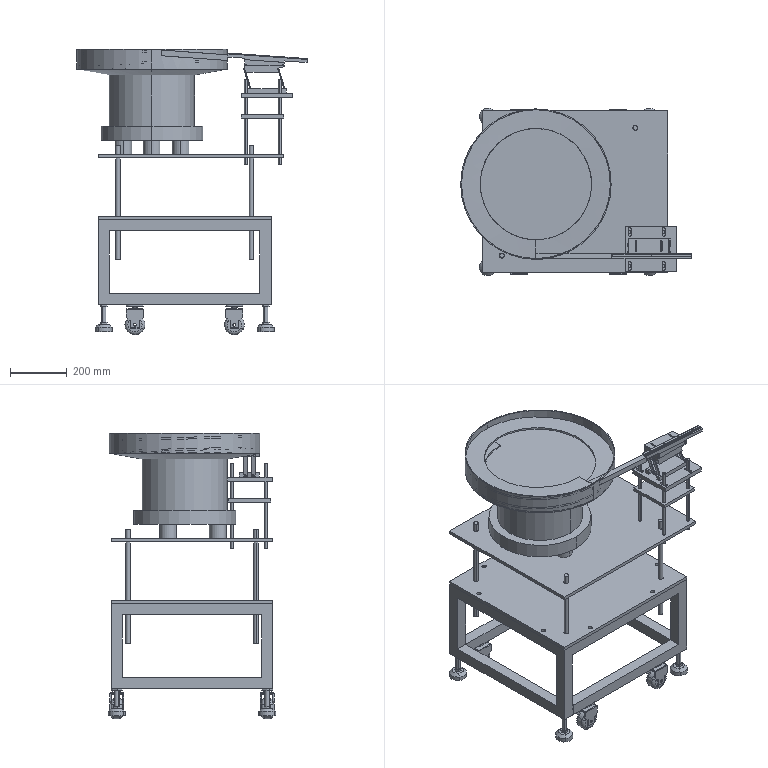Assembly | SolidWorks | mm | 52 component files | 52 solids | 1070 faces | box 812.32 x 590 x 1004.72 mm | volume 42903863 mm3 | plane 672 | cylinder 321 | cone 58 | torus 16 | spline 3 | commonest cylinder face diameters 10 x56 16 x40 10.5 x24 15 x16 9 x16 6.5 x16 3.3 x16 4.5 x16
Bill of materials:
Wheel | 4 |  | Short solid cylinder with large rounded edges on both ends and a small central axial hole.
WheelBracket | 4 |  | U-shaped bent-sheet bracket: a flat rectangular top web with one small hole, and two parallel side flanges folded down. Each flange narrows to a lower tab with one round hole.
WheelRetainingBlock | 4 |  | Flat plate shaped like a rectangle with rounded ends. It has one larger central hole and two smaller holes, one at each end on the long axis, plus a protrusion on the underside with a curved/tapered profile.
WheelRetainingPin | 4 |  | Plain solid cylinder with small chamfers on both end edges.
FootPad | 4 |  | Turned part: a slender cylindrical shaft rising from a larger short cylindrical base. The base has a conical chamfer between its outer edge and the shaft.
FootPadScrew | 8 |  | Hexagonal ring/nut-like body with a large round central bore and chamfered corners on both faces.
Frame01-1 | 1 |  | Open rectangular box frame made of square-section members along all twelve edges of a rectangular prism.
CSFA2082 072 | 1 |  | Thin flat rectangular (near-square) plate with twelve through holes around the perimeter: four larger holes inset at the corners and eight smaller holes in pairs along each edge.
CSFA2082 073 | 1 |  | Thin flat rectangular plate with four larger holes near the corners and four smaller holes in a square pattern around one of the corner holes.
CSFA2082 074 | 1 |  | Square flat plate of moderate thickness with four through holes, one inset near each corner.
CSFA2082 076 | 1 |  | Thick rectangular plate with four elongated slots near the corners, all running the same direction, and a faint thin L-shaped line or groove on the top face.
CSFA2082 077 | 1 |  | Rectangular block shaped like a wedge, with a top face sloping along its length. It has four larger holes at the corners and four smaller holes inboard in two pairs.
CSFA2082 078-1 | 4 |  | Long, slender, straight solid-looking cylindrical rod with flat ends.
CSFA2082 078 | 4 |  | Long, slender, straight cylindrical rod with flat ends, nearly identical to unnamed part but slightly thicker relative to its length.
CSFA2082 079 | 1 |  | Long, narrow base strip with a wider rectangular plate section in the middle on one side. A lengthwise rectangular channel runs along the strip, the plate section has two parallel elongated slots, and small round holes are spaced along the strip.
FeedingPressureBlock | 2 |  | Thin, flat rectangular bar with two round holes spaced along its length.
Part77 | 1 |  | Rectangular block or plate with angled long side faces and a notched, angled profile at one end. Several round holes are grouped near each short end, with one near the centre.
Part78 | 1 |  | Thick rectangular plate with a rectangular notch centred in each short end, leaving four corner ears. Each ear has one round hole.
Part79 | 4 |  | Flat rectangular link bar with square ends and one round hole near each end.
PlasticVibratoryFeederCSFA2082 | 1 |  | Rotationally symmetric part: a large disc head with a conical underside, a narrower cylindrical body, a flange ring below, and small cylindrical pins sticking out of the bottom. A shallow circular groove is on the top face, and a thin radial strip or tab extends past the head's rim.
Mates:
1. concentric | CSFA2082 072-1 face at (132.551, 208.824, 240) dir (0, 0, 1) r 8.5 | CSFA2082 073-1 face at (132.551, 208.824, 457) dir (0, 0, 1) r 9
2. distance | CSFA2082 072-1 face at (202.551, 268.824, 240) dir (0, 0, 1) | CSFA2082 073-1 face at (247.551, 268.824, 445) dir (0, 0, -1)
3. coincident | CSFA2082 073-1 face at (247.551, 268.824, 457) dir (0, 0, 1) | PlasticVibratoryFeederCSFA2082-1 face at (-217.593, -107.346, 457) dir (0, 0, -1)
4. distance | CSFA2082 074-1 face at (247.551, -143.176, 585) dir (0, 0, -1) | CSFA2082 073-1 face at (247.551, 268.824, 457) dir (0, 0, 1)
5. coincident | CSFA2082 076-1 face at (277.301, -138.176, 673) dir (0, 0, 1) | FlatFeed-1/Part78-1 face at (256.301, -253.176, 673) dir (0, 0, -1)
6. coincident | FlatFeed-1/Part77-1 face at (248.594, -253.176, 771) dir (0, 0, 1) | CSFA2082 077-1 face at (248.594, -183.176, 771) dir (0, 0, -1)
7. concentric | CSFA2082 073-1 face at (132.551, -241.176, 457) dir (0, 0, 1) r 9 | CSFA2082 078-6 face at (132.551, -241.176, 487) dir (0, 0, -1) r 8
8. concentric | CSFA2082 073-1 face at (-337.449, -241.176, 457) dir (0, 0, 1) r 9 | CSFA2082 078-5 face at (-337.449, -241.176, 487) dir (0, 0, -1) r 8
9. concentric | CSFA2082 073-1 face at (-337.449, 208.824, 457) dir (0, 0, 1) r 9 | CSFA2082 078-9 face at (-337.449, 208.824, 487) dir (0, 0, -1) r 8
10. concentric | CSFA2082 073-1 face at (132.551, 208.824, 457) dir (0, 0, 1) r 9 | CSFA2082 078-7 face at (132.551, 208.824, 487) dir (0, 0, -1) r 8
11. coincident | CSFA2082 078-5 face at (-337.449, -241.176, 487) dir (0, 0, 1) | CSFA2082 078-6 face at (132.551, -241.176, 487) dir (0, 0, 1)
12. coincident | CSFA2082 078-5 face at (-337.449, -241.176, 487) dir (0, 0, 1) | CSFA2082 078-9 face at (-337.449, 208.824, 487) dir (0, 0, 1)
13. coincident | CSFA2082 078-5 face at (-337.449, -241.176, 487) dir (0, 0, 1) | CSFA2082 078-7 face at (132.551, 208.824, 487) dir (0, 0, 1)
14. coincident | CSFA2082 072-1 face at (202.551, 268.824, 228) dir (0, 0, -1) | AssemblyVibratoryFeederChassis-1/Frame01-1-1 face at (-407.449, 268.824, 228) dir (0, 0, 1)
15. concentric | CSFA2082 072-1 face at (-337.449, -241.176, 240) dir (0, 0, 1) r 8.5 | CSFA2082 078-5 face at (-337.449, -241.176, 487) dir (0, 0, -1) r 8
16. concentric | CSFA2082 073-1 face at (112.551, -278.176, 457) dir (0, 0, 1) r 5.25 | CSFA2082 078-1-1 face at (112.551, -278.176, 720) dir (0, 0, -1) r 5
17. concentric | CSFA2082 074-1 face at (112.551, -278.176, 597) dir (0, 0, 1) r 5.25 | CSFA2082 078-1-1 face at (112.551, -278.176, 720) dir (0, 0, -1) r 5
18. distance | CSFA2082 078-1-1 face at (112.551, -278.176, 420) dir (0, 0, -1) | CSFA2082 073-1 face at (247.551, 268.824, 445) dir (0, 0, -1)
19. concentric | CSFA2082 073-1 face at (232.551, -278.176, 457) dir (0, 0, 1) r 5.25 | CSFA2082 078-1-2 face at (232.551, -278.176, 720) dir (0, 0, -1) r 5
20. coincident | CSFA2082 078-1-1 face at (112.551, -278.176, 420) dir (0, 0, -1) | CSFA2082 078-1-2 face at (232.551, -278.176, 420) dir (0, 0, -1)
21. coincident | CSFA2082 078-1-2 face at (232.551, -278.176, 420) dir (0, 0, -1) | CSFA2082 078-1-4 face at (232.551, -158.176, 420) dir (0, 0, -1)
22. coincident | CSFA2082 078-1-3 face at (112.551, -158.176, 420) dir (0, 0, -1) | CSFA2082 078-1-4 face at (232.551, -158.176, 420) dir (0, 0, -1)
23. concentric | CSFA2082 073-1 face at (112.551, -158.176, 457) dir (0, 0, 1) r 5.25 | CSFA2082 078-1-3 face at (112.551, -158.176, 720) dir (0, 0, -1) r 5
24. concentric | CSFA2082 073-1 face at (232.551, -158.176, 457) dir (0, 0, 1) r 5.25 | CSFA2082 078-1-4 face at (232.551, -158.176, 720) dir (0, 0, -1) r 5
25. tangent | CSFA2082 076-1 face at (117.551, -268.176, 657) dir (-1, 0, 0) | CSFA2082 078-1-1 face at (112.551, -278.176, 720) dir (0, 0, -1) r 5
26. tangent | CSFA2082 076-1 face at (237.551, -268.176, 657) dir (-1, 0, 0) | CSFA2082 078-1-2 face at (232.551, -278.176, 720) dir (0, 0, -1) r 5
27. distance | CSFA2082 076-1 face at (97.301, -298.176, 673) dir (0, -1, 0) | CSFA2082 074-1 face at (97.551, -293.176, 597) dir (0, -1, 0)
28. distance | FlatFeed-1/Part78-1 face at (256.301, -253.176, 673) dir (0, -1, 0) | CSFA2082 076-1 face at (97.301, -298.176, 673) dir (0, -1, 0)
29. distance | CSFA2082 078-9 face at (-337.449, 208.824, 487) dir (0, 0, 1) | CSFA2082 073-1 face at (247.551, 268.824, 457) dir (0, 0, 1)
30. coincident | CSFA2082 079-1 face at (329.522, -253.176, 791.691) dir (0.06976, 0, 0.9976) | FeedingPressureBlock-1 face at (50.204, -233.176, 811.222) dir (-0.06976, 0, -0.9976)
31. concentric | CSFA2082 079-1 face at (85.119, -236.676, 808.781) dir (0.06976, 0, 0.9976) r 1.65 | FeedingPressureBlock-1 face at (85.328, -236.676, 811.774) dir (-0.06976, 0, -0.9976) r 2.25
32. concentric | CSFA2082 079-1 face at (154.949, -236.676, 803.898) dir (0.06976, 0, 0.9976) r 1.65 | FeedingPressureBlock-1 face at (155.158, -236.676, 806.891) dir (-0.06976, 0, -0.9976) r 2.25
33. distance | FlatFeed-1/Part78-1 face at (256.301, -253.176, 688) dir (1, 0, 0) | CSFA2082 076-1 face at (277.301, -298.176, 673) dir (1, 0, 0)
34. coincident | CSFA2082 079-1 face at (329.522, -253.176, 791.691) dir (0.06976, 0, 0.9976) | FeedingPressureBlock-2 face at (329.522, -233.176, 791.691) dir (-0.06976, 0, -0.9976)
35. concentric | CSFA2082 079-1 face at (224.778, -236.676, 799.015) dir (0.06976, 0, 0.9976) r 1.65 | FeedingPressureBlock-2 face at (224.778, -236.676, 799.015) dir (0.06976, 0, 0.9976) r 2.25
36. concentric | CSFA2082 079-1 face at (294.608, -236.676, 794.132) dir (0.06976, 0, 0.9976) r 1.65 | FeedingPressureBlock-2 face at (294.608, -236.676, 794.132) dir (0.06976, 0, 0.9976) r 2.25
37. coincident | PlasticVibratoryFeederCSFA2082-1 face at (-217.593, -253.176, 507) dir (0, -1, 0) | CSFA2082 079-1 face at (248.943, -253.176, 786.198) dir (0, -1, 0)
38. coincident | FlatFeed-1/Part77-1 face at (108.594, -253.176, 771) dir (-1, 0, 0) | CSFA2082 077-1 face at (108.594, -253.176, 791) dir (-1, 0, 0)
39. coincident | FlatFeed-1/Part77-1 face at (117.647, -253.176, 730.745) dir (0, -1, 0) | CSFA2082 077-1 face at (108.594, -253.176, 791) dir (0, -1, 0)
40. coincident | CSFA2082 077-1 face at (108.594, -119.176, 791) dir (0.06976, 0, 0.9976) | CSFA2082 079-1 face at (108.935, -253.176, 790.976) dir (-0.06976, 0, -0.9976)
41. distance | CSFA2082 074-1 face at (247.551, -143.176, 597) dir (0, 0, 1) | CSFA2082 076-1 face at (277.301, -138.176, 657) dir (0, 0, -1)
42. coincident | CSFA2082 077-1 face at (108.594, -253.176, 791) dir (0, -1, 0) | CSFA2082 079-1 face at (248.943, -253.176, 786.198) dir (0, -1, 0)
43. coincident | CSFA2082 077-1 face at (248.594, -253.176, 791) dir (1, 0, 0) | CSFA2082 079-1 edge at (248.594, -253.176, 781.21) dir (0, 1, 0)
44. concentric | Frame01-1-1 face at (-301.003, -194.728, 280) dir (0, -1, 0) r 8 | FootPad-1 face at (-301.003, -164.728, 280) dir (0, -1, 0) r 8
45. distance | FootPad-1 face at (-301.003, -264.728, 280) dir (0, 1, 0) | Frame01-1-1 face at (-321.003, -194.728, -270) dir (0, -1, 0)
46. concentric | Frame01-1-1 face at (-301.003, -194.728, -250) dir (0, -1, 0) r 8 | FootPad-2 face at (-301.003, -164.728, -250) dir (0, -1, 0) r 8
47. coincident | FootPad-1 face at (-301.003, -289.728, 280) dir (0, -1, 0) | FootPad-2 face at (-301.003, -289.728, -250) dir (0, -1, 0)
48. coincident | FootPad-1 face at (-301.003, -289.728, 280) dir (0, -1, 0) | FootPad-3 face at (268.997, -289.728, 280) dir (0, -1, 0)
49. coincident | FootPad-3 face at (268.997, -289.728, 280) dir (0, -1, 0) | FootPad-4 face at (268.997, -289.728, -250) dir (0, -1, 0)
50. concentric | Frame01-1-1 face at (268.997, -194.728, 280) dir (0, -1, 0) r 8 | FootPad-3 face at (268.997, -164.728, 280) dir (0, -1, 0) r 8
51. concentric | Frame01-1-1 face at (268.997, -194.728, -250) dir (0, -1, 0) r 8 | FootPad-4 face at (268.997, -164.728, -250) dir (0, -1, 0) r 8
52. coincident | Frame01-1-1 face at (288.997, -194.728, 300) dir (0, 0, 1) | AssemblyWheel-1/WheelRetainingBlock-1 face at (-221.003, -194.728, 300) dir (0, 0, 1)
53. coincident | Frame01-1-1 face at (-321.003, -194.728, -270) dir (0, -1, 0) | AssemblyWheel-1/WheelRetainingBlock-1 face at (-221.003, -194.728, 300) dir (0, 1, 0)
54. distance | Frame01-1-1 face at (-321.003, 105.272, -270) dir (-1, 0, 0) | AssemblyWheel-1/WheelBracket-1 face at (-221.003, -278.449, 305) dir (-1, 0, 0)
55. coincident | AssemblyWheel-1/WheelRetainingBlock-1 face at (-221.003, -194.728, 300) dir (0, 0, 1) | AssemblyWheel-2/WheelRetainingBlock-1 face at (128.997, -194.728, 300) dir (0, 0, 1)
56. coincident | AssemblyWheel-1/WheelBracket-1 face at (-221.003, -209.728, 305) dir (0, 1, 0) | AssemblyWheel-2/WheelBracket-1 face at (128.997, -209.728, 305) dir (0, 1, 0)
57. coincident | AssemblyWheel-2/WheelBracket-1 face at (128.997, -209.728, 305) dir (0, 1, 0) | AssemblyWheel-4/WheelBracket-1 face at (128.997, -209.728, -225) dir (0, 1, 0)
58. coincident | AssemblyWheel-1/WheelBracket-1 face at (-221.003, -209.728, 305) dir (0, 1, 0) | AssemblyWheel-3/WheelBracket-1 face at (-221.003, -209.728, -225) dir (0, 1, 0)
59. distance | AssemblyWheel-2/WheelBracket-1 face at (188.997, -278.449, 305) dir (1, 0, 0) | Frame01-1-1 face at (288.997, 105.272, -270) dir (1, 0, 0)
60. coincident | Frame01-1-1 face at (288.997, -194.728, -270) dir (0, 0, -1) | AssemblyWheel-4/WheelRetainingBlock-1 face at (128.997, -194.728, -270) dir (0, 0, -1)
61. coincident | Frame01-1-1 face at (288.997, -194.728, -270) dir (0, 0, -1) | AssemblyWheel-3/WheelRetainingBlock-1 face at (-221.003, -194.728, -270) dir (0, 0, -1)
62. coincident | AssemblyWheel-2/WheelBracket-1 face at (188.997, -278.449, 305) dir (1, 0, 0) | AssemblyWheel-4/WheelBracket-1 face at (188.997, -278.449, -225) dir (1, 0, 0)
63. coincident | AssemblyWheel-1/WheelBracket-1 face at (-221.003, -278.449, 305) dir (-1, 0, 0) | AssemblyWheel-3/WheelBracket-1 face at (-221.003, -278.449, -225) dir (-1, 0, 0)
64. concentric | FootPad-1 face at (-301.003, -164.728, 280) dir (0, -1, 0) r 8 | FootPadScrew-1 face at (-301.003, -256.728, 280) dir (0, 1, 0) r 8
65. coincident | FootPad-1 face at (-301.003, -264.728, 280) dir (0, 1, 0) | FootPadScrew-1 face at (-288.503, -264.728, 280) dir (0, -1, 0)
66. concentric | FootPad-1 face at (-301.003, -164.728, 280) dir (0, -1, 0) r 8 | FootPadScrew-2 face at (-301.003, -194.728, 280) dir (0, 1, 0) r 8
67. parallel | Frame01-1-1 face at (288.997, -194.728, 300) dir (0, 0, 1) | FootPadScrew-2 face at (-307.253, -194.728, 290.825) dir (0, 0, 1)
68. coincident | FootPadScrew-1 face at (-307.253, -256.728, 290.825) dir (0, 0, 1) | FootPadScrew-2 face at (-307.253, -194.728, 290.825) dir (0, 0, 1)
69. coincident | Frame01-1-1 face at (-321.003, -194.728, -270) dir (0, -1, 0) | FootPadScrew-2 face at (-288.503, -194.728, 280) dir (0, 1, 0)
70. concentric | FootPad-3 face at (268.997, -164.728, 280) dir (0, -1, 0) r 8 | FootPadScrew-5 face at (268.997, -256.728, 280) dir (0, 1, 0) r 8
71. concentric | FootPad-3 face at (268.997, -164.728, 280) dir (0, -1, 0) r 8 | FootPadScrew-6 face at (268.997, -194.728, 280) dir (0, 1, 0) r 8
72. coincident | FootPad-3 face at (268.997, -264.728, 280) dir (0, 1, 0) | FootPadScrew-5 face at (281.497, -264.728, 280) dir (0, -1, 0)
73. coincident | Frame01-1-1 face at (-321.003, -194.728, -270) dir (0, -1, 0) | FootPadScrew-6 face at (281.497, -194.728, 280) dir (0, 1, 0)
74. coincident | FootPadScrew-2 face at (-307.253, -194.728, 290.825) dir (0, 0, 1) | FootPadScrew-6 face at (262.747, -194.728, 290.825) dir (0, 0, 1)
75. coincident | FootPadScrew-5 face at (262.747, -256.728, 290.825) dir (0, 0, 1) | FootPadScrew-6 face at (262.747, -194.728, 290.825) dir (0, 0, 1)
76. concentric | FootPad-4 face at (268.997, -164.728, -250) dir (0, -1, 0) r 8 | FootPadScrew-8 face at (268.997, -194.728, -250) dir (0, 1, 0) r 8
77. concentric | FootPad-4 face at (268.997, -164.728, -250) dir (0, -1, 0) r 8 | FootPadScrew-7 face at (268.997, -256.728, -250) dir (0, 1, 0) r 8
78. coincident | FootPad-4 face at (268.997, -264.728, -250) dir (0, 1, 0) | FootPadScrew-7 face at (281.497, -264.728, -250) dir (0, -1, 0)
79. coincident | Frame01-1-1 face at (-321.003, -194.728, -270) dir (0, -1, 0) | FootPadScrew-8 face at (275.247, -194.728, -260.825) dir (0, 1, 0)
80. parallel | Frame01-1-1 face at (288.997, -194.728, -270) dir (0, 0, -1) | FootPadScrew-8 face at (275.247, -194.728, -260.825) dir (0, 0, -1)
81. coincident | FootPadScrew-7 face at (275.247, -256.728, -260.825) dir (0, 0, -1) | FootPadScrew-8 face at (275.247, -194.728, -260.825) dir (0, 0, -1)
82. concentric | FootPad-2 face at (-301.003, -164.728, -250) dir (0, -1, 0) r 8 | FootPadScrew-4 face at (-301.003, -194.728, -250) dir (0, 1, 0) r 8
83. concentric | FootPad-2 face at (-301.003, -164.728, -250) dir (0, -1, 0) r 8 | FootPadScrew-3 face at (-301.003, -256.728, -250) dir (0, 1, 0) r 8
84. coincident | FootPad-2 face at (-301.003, -264.728, -250) dir (0, 1, 0) | FootPadScrew-3 face at (-288.503, -264.728, -250) dir (0, -1, 0)
85. coincident | Frame01-1-1 face at (-321.003, -194.728, -270) dir (0, -1, 0) | FootPadScrew-4 face at (-288.503, -194.728, -250) dir (0, 1, 0)
86. coincident | FootPadScrew-3 face at (-294.753, -256.728, -260.825) dir (0, 0, -1) | FootPadScrew-7 face at (275.247, -256.728, -260.825) dir (0, 0, -1)
87. coincident | FootPadScrew-3 face at (-294.753, -256.728, -260.825) dir (0, 0, -1) | FootPadScrew-4 face at (-294.753, -194.728, -260.825) dir (0, 0, -1)
88. concentric | WheelBracket-1 face at (27.751, -15.353, 0) dir (-1, 0, 0) r 5 | Wheel-1 face at (22.751, -15.353, 0) dir (-1, 0, 0) r 5
89. coincident | WheelBracket-1 face at (22.751, 35.368, -30) dir (-1, 0, 0) | Wheel-1 face at (22.751, -15.353, 0) dir (1, 0, 0)
90. concentric | WheelBracket-1 face at (2.751, -28.353, 0) dir (0, 1, 0) r 5 | WheelRetainingPin-1 face at (2.751, 35.368, 0) dir (0, 1, 0) r 5
91. coincident | WheelBracket-1 face at (-17.249, 35.368, -30) dir (0, -1, 0) | WheelRetainingPin-1 face at (2.751, 35.368, 0) dir (0, -1, 0)
92. concentric | WheelRetainingPin-1 face at (2.751, 35.368, 0) dir (0, 1, 0) r 5 | WheelRetainingBlock-1 face at (2.751, 43.031, 0) dir (0, 1, 0) r 5
93. coincident | WheelRetainingPin-1 face at (2.751, 55.368, 0) dir (0, 1, 0) | WheelRetainingBlock-1 face at (-17.249, 55.368, -30) dir (0, 1, 0)
94. parallel | WheelBracket-1 face at (27.751, 40.368, -30) dir (1, 0, 0) | WheelRetainingBlock-1 face at (22.751, 55.368, -30) dir (1, 0, 0)
95. coincident | Part78-1 face at (-99.502, -23.554, 62.5) dir (0, 0, 1) | Part77-1 face at (39.152, 34.191, 62.5) dir (0, 0, 1)
96. coincident | Part77-1 face at (48.205, 63.801, -7.5) dir (0.9563, -0.2924, 0) | Part79-3 face at (21.498, -23.554, 7.5) dir (-0.9563, 0.2924, 0)
97. coincident | Part77-1 face at (48.205, 63.801, -7.5) dir (0.9563, -0.2924, 0) | Part79-4 face at (21.498, -23.554, 35.5) dir (-0.9563, 0.2924, 0)
98. distance | Part77-1 face at (-91.795, 74.446, -7.5) dir (0, 1, 0) | Part78-1 face at (-99.502, -23.554, -7.5) dir (0, -1, 0)
99. coincident | Part78-1 face at (21.498, -23.554, 7.5) dir (0.9563, -0.2924, 0) | Part77-1 face at (48.205, 63.801, -7.5) dir (0.9563, -0.2924, 0)
100. coincident | Part78-1 face at (-95.502, -23.554, 7.5) dir (-0.9563, 0.2924, 0) | Part79-1 face at (-95.502, -23.554, 7.5) dir (0.9563, -0.2924, 0)
101. coincident | Part78-1 face at (-95.502, -23.554, 7.5) dir (-0.9563, 0.2924, 0) | Part79-2 face at (-95.502, -23.554, 35.5) dir (0.9563, -0.2924, 0)
102. coincident | Part79-1 face at (-98.371, -22.677, 19.5) dir (-0.2924, -0.9563, 0) | Part79-2 face at (-98.371, -22.677, 47.5) dir (-0.2924, -0.9563, 0)
103. coincident | Part78-1 edge at (-95.502, -23.554, 7.5) dir (0, 0, 1) | Part79-2 edge at (-95.502, -23.554, 35.5) dir (0, 0, 1)
104. coincident | Part78-1 face at (21.498, -23.554, 7.5) dir (0.9563, -0.2924, 0) | Part79-3 face at (21.498, -23.554, 7.5) dir (-0.9563, 0.2924, 0)
105. coincident | Part78-1 edge at (21.498, -23.554, 7.5) dir (0, 0, 1) | Part79-3 edge at (21.498, -23.554, 7.5) dir (0, 0, 1)
106. coincident | Part79-3 edge at (24.367, -24.431, 7.5) dir (0, 0, 1) | Part79-4 edge at (24.367, -24.431, 35.5) dir (0, 0, 1)
107. coincident | Part78-1 face at (54.358, 4.765, 47.5) dir (0, 0, -1) | Part79-4 face at (48.192, 63.757, 47.5) dir (0, 0, 1)
108. coincident | Part78-1 face at (54.358, 4.765, 7.5) dir (0, 0, 1) | Part79-3 face at (48.192, 63.757, 7.5) dir (0, 0, -1)
109. coincident | Part78-1 face at (-99.502, -23.554, 7.5) dir (0, 0, 1) | Part79-1 face at (-71.677, 64.634, 7.5) dir (0, 0, -1)
110. coincident | Part78-1 face at (-99.502, -23.554, 47.5) dir (0, 0, -1) | Part79-2 face at (-71.677, 64.634, 47.5) dir (0, 0, 1)